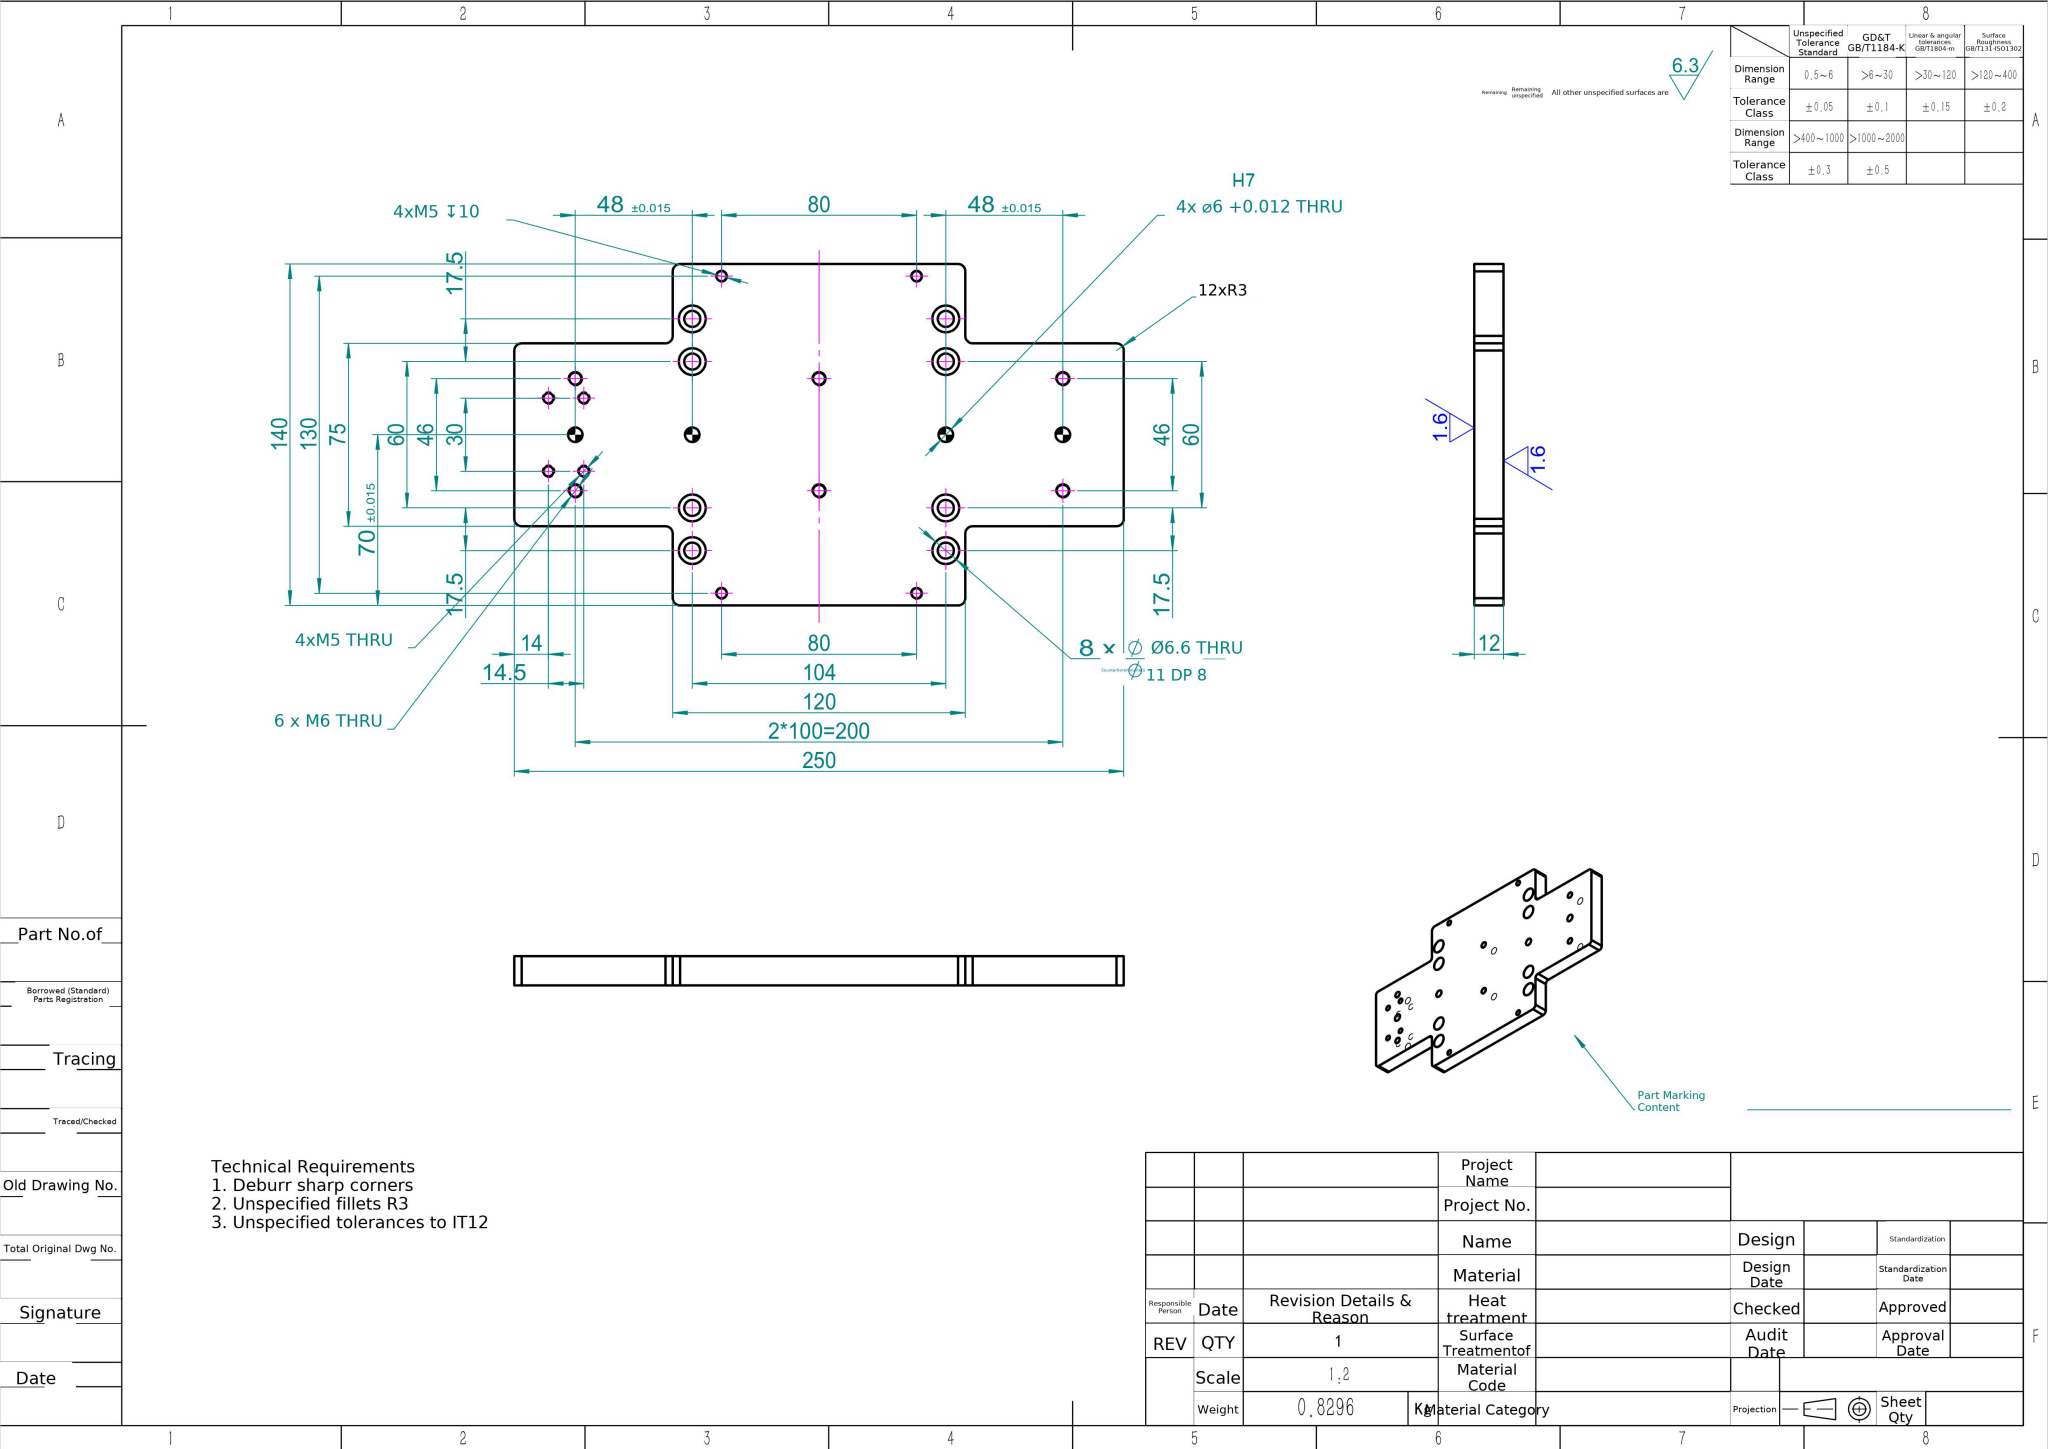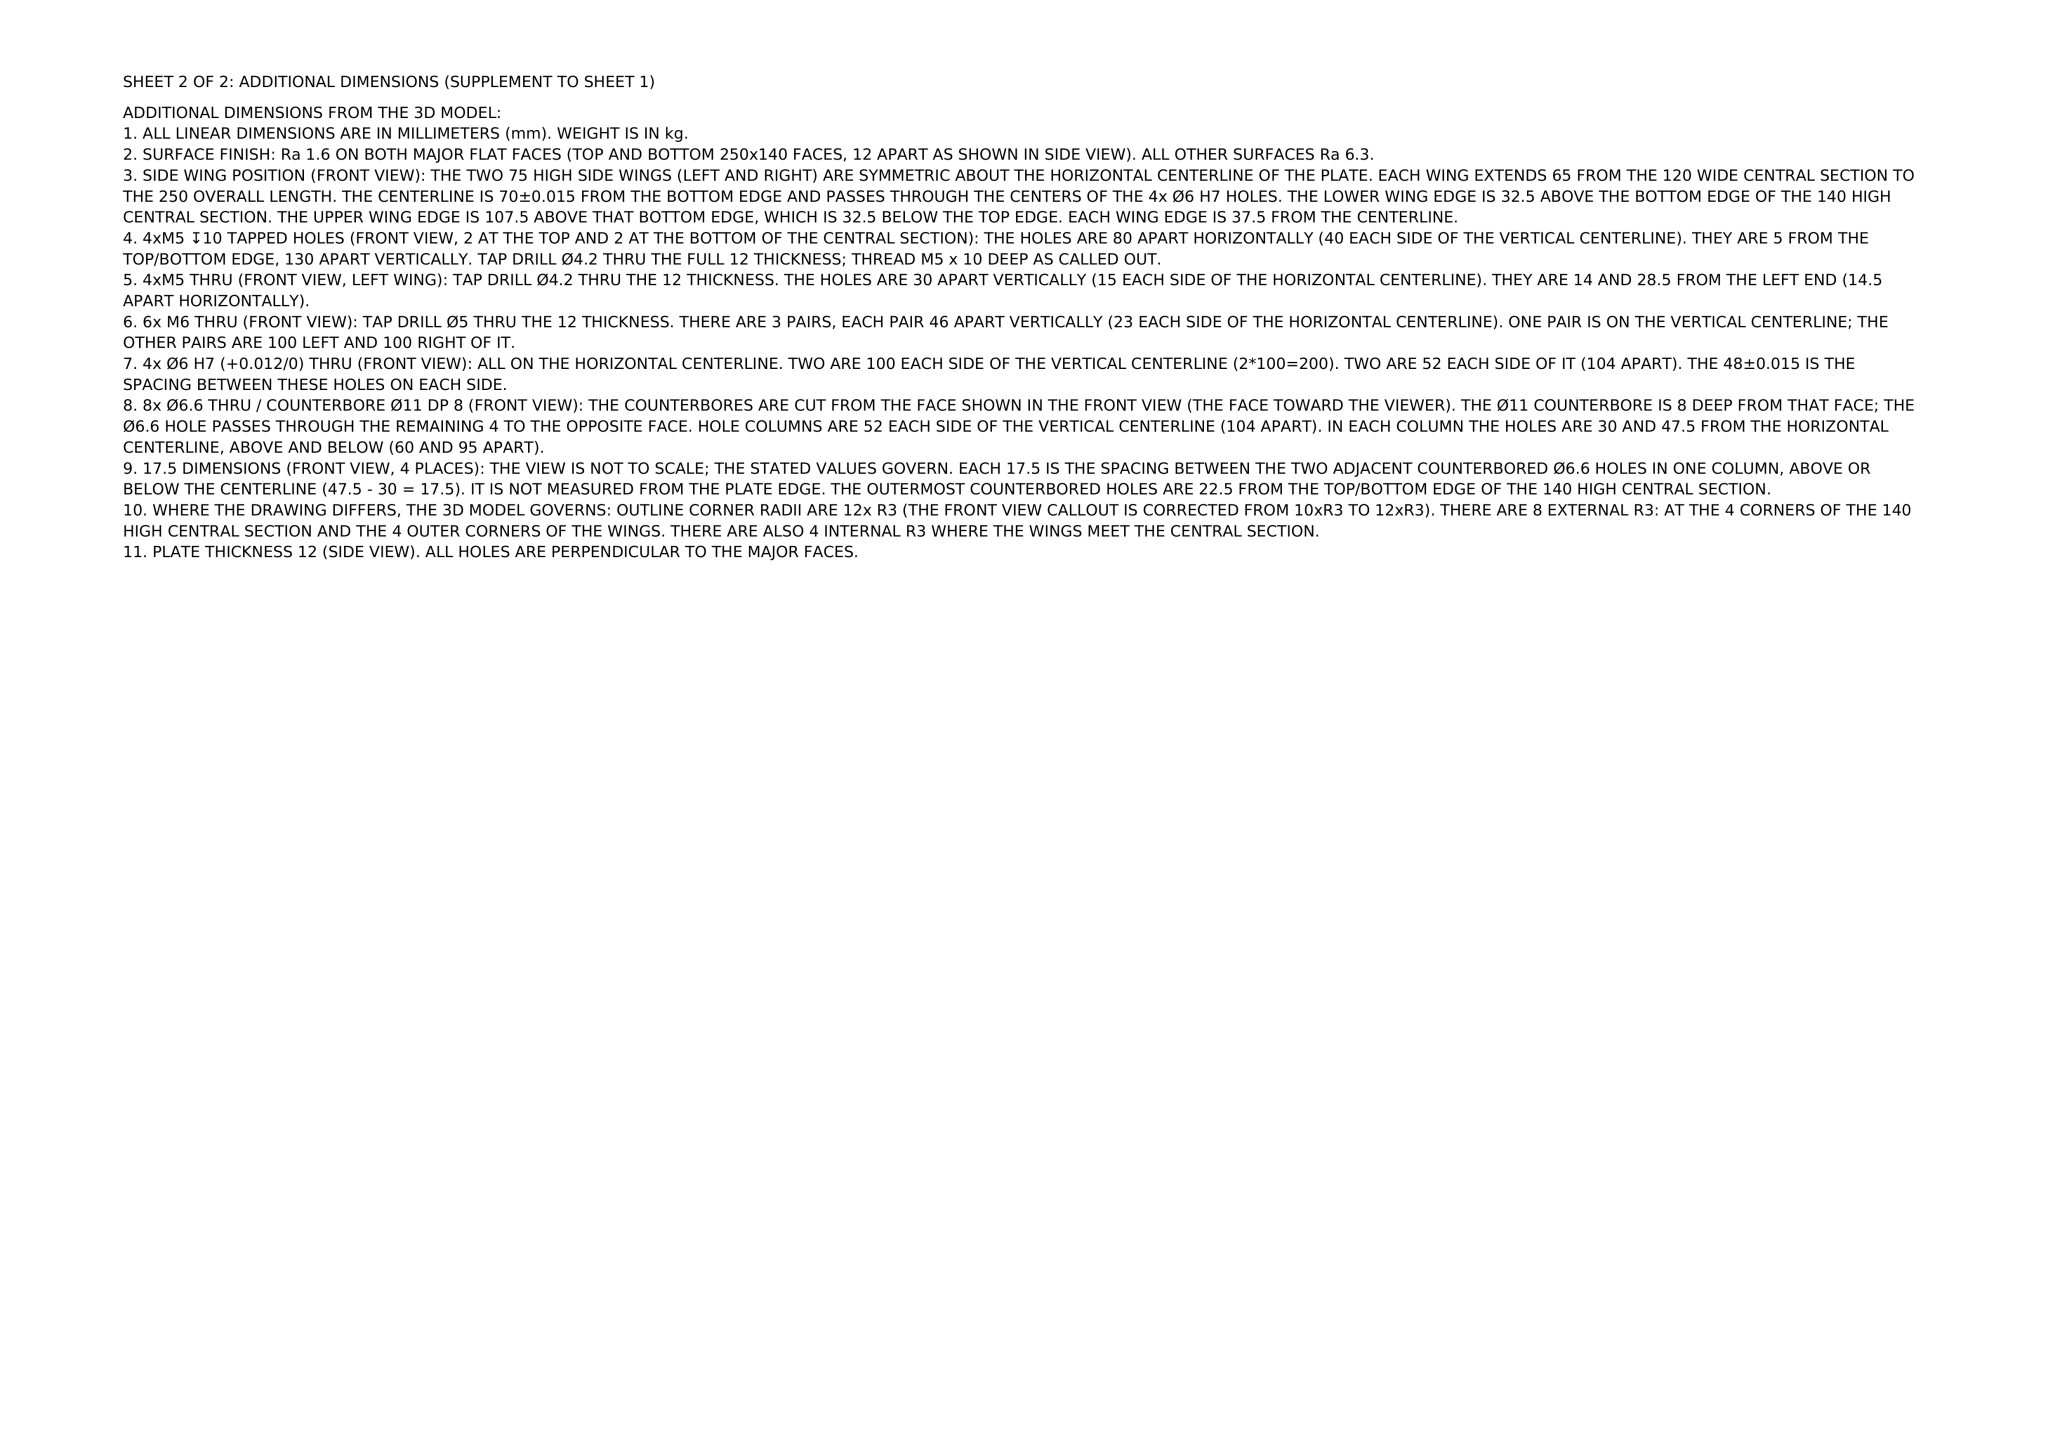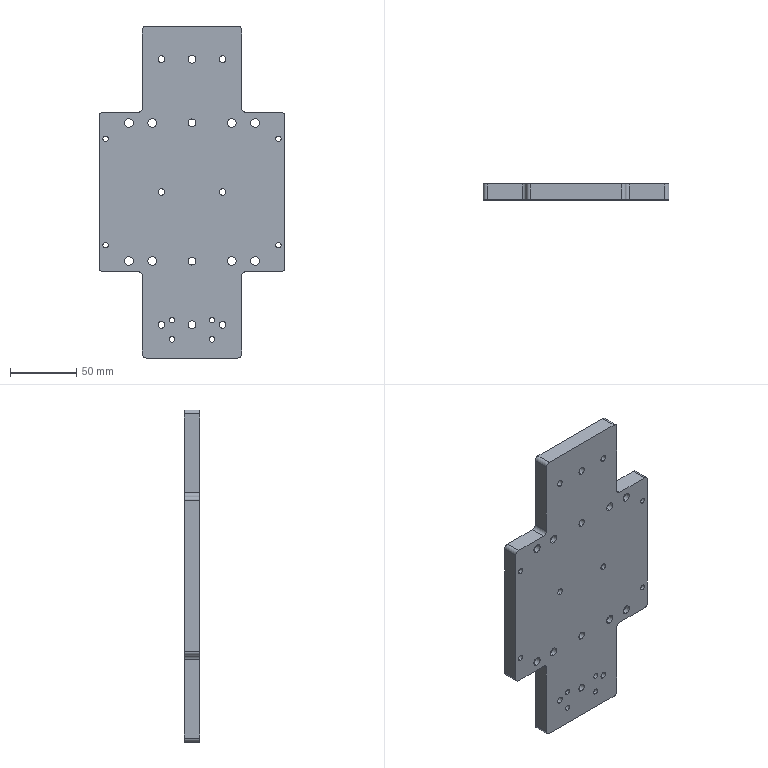Part | NX | mm | 1 solid | 102 faces | box 140 x 12 x 250 mm | volume 307270 mm3 | cylinder 80 | plane 22 | commonest cylinder face diameters 6 x20 4.2 x16 11 x16 6.6 x16 5 x12